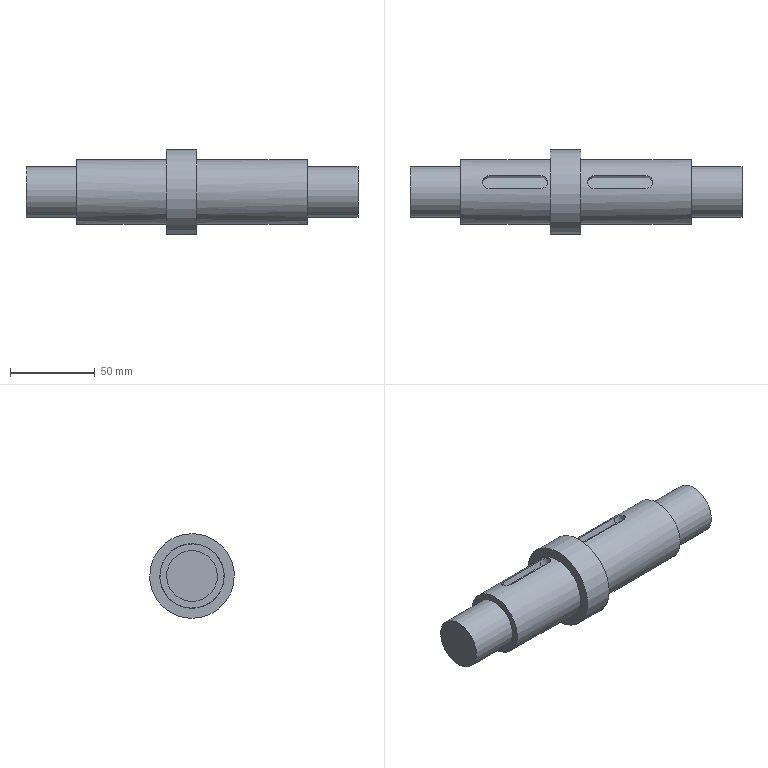Component | NX | CHUANDONGZHOU | 1 solid | 21 faces | volume 209303 mm3 | plane 12 | cylinder 9 | commonest cylinder face diameters 8 x4 38 x2 30 x2 50 x1